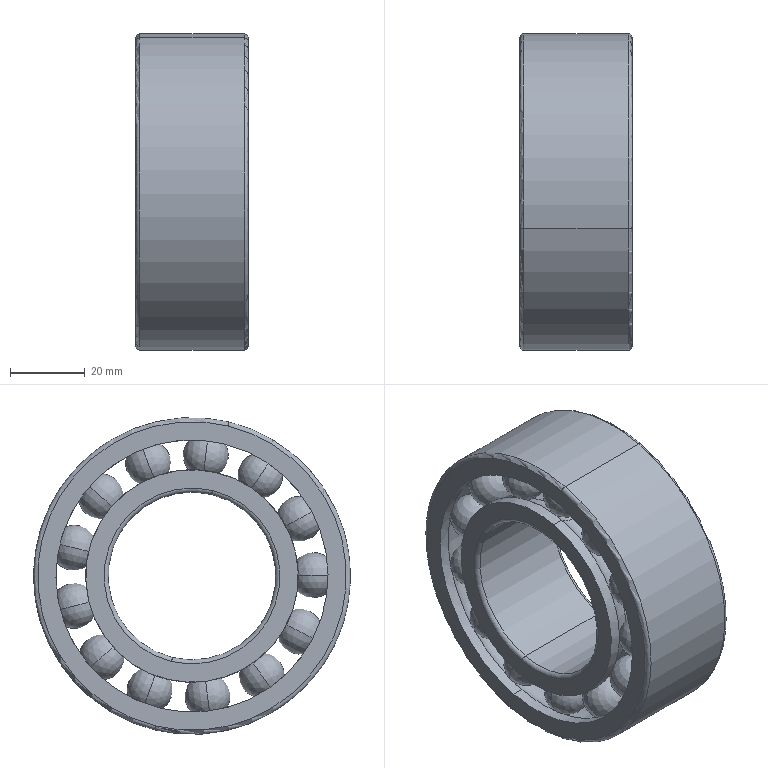Component | SolidWorks | 9DoubleRowAngularContactBallBearing[GBT296-2015][3209A]-1 | 1 solid | 166 faces | volume 85822 mm3 | torus 98 | sphere 52 | cylinder 12 | plane 4 | commonest cylinder face diameters 57 x4 73 x4 45 x2 85 x2 | material GCr4